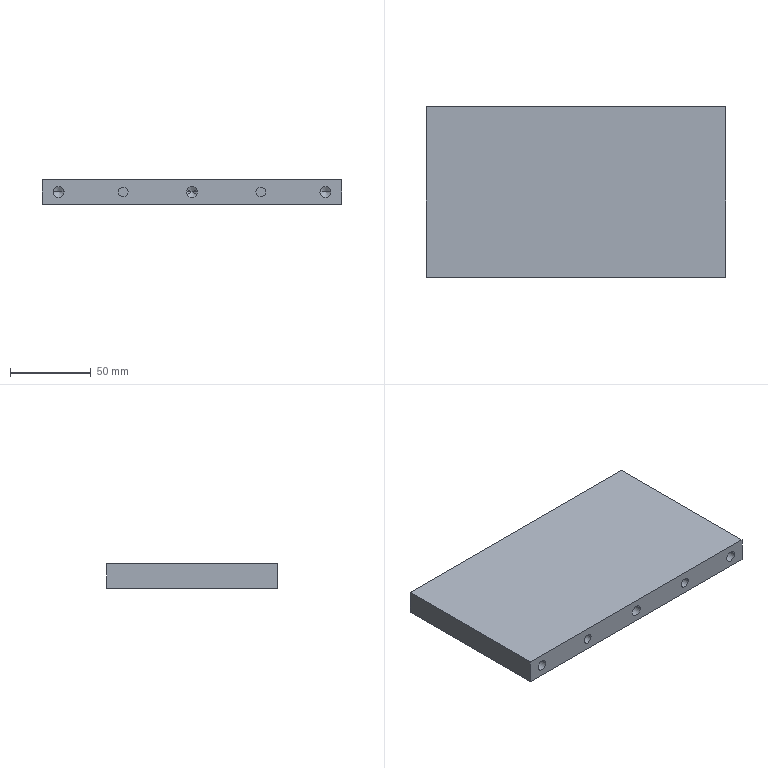Component | SolidWorks | FlipMechanismB-10-1 | 1 solid | 42 faces | box 185 x 105.4 x 15 mm | volume 286584 mm3 | cylinder 20 | cone 12 | plane 10 | commonest cylinder face diameters 6.8 x12 6 x8
STEP:
#1=CARTESIAN_POINT('',(-2.677,-1.323,1.555));
#2=VERTEX_POINT('',#1);
#3=CARTESIAN_POINT('',(-2.441,-1.323,1.555));
#4=VERTEX_POINT('',#3);
#5=CARTESIAN_POINT('',(-2.559,-1.323,1.555));
#6=DIRECTION('',(-0.,-1.,0.));
#7=DIRECTION('',(1.,0.,0.));
#8=AXIS2_PLACEMENT_3D('',#5,#6,#7);
#9=CIRCLE('',#8,0.1181);
#10=EDGE_CURVE('',#2,#4,#9,.T.);
#11=ORIENTED_EDGE('',*,*,#10,.F.);
#12=CARTESIAN_POINT('',(-2.677,-1.559,1.555));
#13=VERTEX_POINT('',#12);
#14=CARTESIAN_POINT('',(-2.677,-1.323,1.555));
#15=DIRECTION('',(-0.,-1.,0.));
#16=VECTOR('',#15,39.37);
#17=LINE('',#14,#16);
#18=EDGE_CURVE('',#2,#13,#17,.T.);
#19=ORIENTED_EDGE('',*,*,#18,.T.);
#20=CARTESIAN_POINT('',(-2.441,-1.559,1.555));
#21=VERTEX_POINT('',#20);
#22=CARTESIAN_POINT('',(-2.559,-1.559,1.555));
#23=DIRECTION('',(-0.,-1.,0.));
#24=DIRECTION('',(1.,0.,0.));
#25=AXIS2_PLACEMENT_3D('',#22,#23,#24);
#26=CIRCLE('',#25,0.1181);
#27=EDGE_CURVE('',#13,#21,#26,.T.);
#28=ORIENTED_EDGE('',*,*,#27,.T.);
#29=CARTESIAN_POINT('',(-2.441,-1.323,1.555));
#30=DIRECTION('',(-0.,-1.,0.));
#31=VECTOR('',#30,39.37);
#32=LINE('',#29,#31);
#33=EDGE_CURVE('',#4,#21,#32,.T.);
#34=ORIENTED_EDGE('',*,*,#33,.F.);
#35=EDGE_LOOP('',(#11,#19,#28,#34));
#36=FACE_OUTER_BOUND('',#35,.T.);
#37=CARTESIAN_POINT('',(-2.559,-1.323,1.555));
#38=DIRECTION('',(-0.,-1.,0.));
#39=DIRECTION('',(1.,0.,0.));
#40=AXIS2_PLACEMENT_3D('',#37,#38,#39);
#41=CYLINDRICAL_SURFACE('',#40,0.1181);
#42=ADVANCED_FACE('',(#36),#41,.F.);
#43=CARTESIAN_POINT('',(0.6693,-1.323,1.555));
#44=VERTEX_POINT('',#43);
#45=CARTESIAN_POINT('',(0.9055,-1.323,1.555));
#46=VERTEX_POINT('',#45);
#47=CARTESIAN_POINT('',(0.7874,-1.323,1.555));
#48=DIRECTION('',(-0.,-1.,0.));
#49=DIRECTION('',(1.,0.,0.));
#50=AXIS2_PLACEMENT_3D('',#47,#48,#49);
#51=CIRCLE('',#50,0.1181);
#52=EDGE_CURVE('',#44,#46,#51,.T.);
#53=ORIENTED_EDGE('',*,*,#52,.F.);
#54=CARTESIAN_POINT('',(0.6693,-1.559,1.555));
#55=VERTEX_POINT('',#54);
#56=CARTESIAN_POINT('',(0.6693,-1.323,1.555));
#57=DIRECTION('',(-0.,-1.,0.));
#58=VECTOR('',#57,39.37);
#59=LINE('',#56,#58);
#60=EDGE_CURVE('',#44,#55,#59,.T.);
#61=ORIENTED_EDGE('',*,*,#60,.T.);
#62=CARTESIAN_POINT('',(0.9055,-1.559,1.555));
#63=VERTEX_POINT('',#62);
#64=CARTESIAN_POINT('',(0.7874,-1.559,1.555));
#65=DIRECTION('',(-0.,-1.,0.));
#66=DIRECTION('',(1.,0.,0.));
#67=AXIS2_PLACEMENT_3D('',#64,#65,#66);
#68=CIRCLE('',#67,0.1181);
#69=EDGE_CURVE('',#55,#63,#68,.T.);
#70=ORIENTED_EDGE('',*,*,#69,.T.);
#71=CARTESIAN_POINT('',(0.9055,-1.323,1.555));
#72=DIRECTION('',(-0.,-1.,0.));
#73=VECTOR('',#72,39.37);
#74=LINE('',#71,#73);
#75=EDGE_CURVE('',#46,#63,#74,.T.);
#76=ORIENTED_EDGE('',*,*,#75,.F.);
#77=EDGE_LOOP('',(#53,#61,#70,#76));
#78=FACE_OUTER_BOUND('',#77,.T.);
#79=CARTESIAN_POINT('',(0.7874,-1.323,1.555));
#80=DIRECTION('',(-0.,-1.,0.));
#81=DIRECTION('',(1.,0.,0.));
#82=AXIS2_PLACEMENT_3D('',#79,#80,#81);
#83=CYLINDRICAL_SURFACE('',#82,0.1181);
#84=ADVANCED_FACE('',(#78),#83,.F.);
#85=CARTESIAN_POINT('',(2.228,-0.6831,1.555));
#86=VERTEX_POINT('',#85);
#87=CARTESIAN_POINT('',(2.496,-0.6831,1.555));
#88=VERTEX_POINT('',#87);
#89=CARTESIAN_POINT('',(2.362,-0.6831,1.555));
#90=DIRECTION('',(-0.,-1.,0.));
#91=DIRECTION('',(1.,0.,0.));
#92=AXIS2_PLACEMENT_3D('',#89,#90,#91);
#93=CIRCLE('',#92,0.1339);
#94=EDGE_CURVE('',#86,#88,#93,.T.);
#95=ORIENTED_EDGE('',*,*,#94,.F.);
#96=CARTESIAN_POINT('',(2.228,-1.559,1.555));
#97=VERTEX_POINT('',#96);
#98=CARTESIAN_POINT('',(2.228,-1.559,1.555));
#99=DIRECTION('',(-0.,-1.,0.));
#100=VECTOR('',#99,39.37);
#101=LINE('',#98,#100);
#102=EDGE_CURVE('',#86,#97,#101,.T.);
#103=ORIENTED_EDGE('',*,*,#102,.T.);
#104=CARTESIAN_POINT('',(2.496,-1.559,1.555));
#105=VERTEX_POINT('',#104);
#106=CARTESIAN_POINT('',(2.362,-1.559,1.555));
#107=DIRECTION('',(-0.,-1.,0.));
#108=DIRECTION('',(1.,0.,0.));
#109=AXIS2_PLACEMENT_3D('',#106,#107,#108);
#110=CIRCLE('',#109,0.1339);
#111=EDGE_CURVE('',#97,#105,#110,.T.);
#112=ORIENTED_EDGE('',*,*,#111,.T.);
#113=CARTESIAN_POINT('',(2.496,-1.559,1.555));
#114=DIRECTION('',(-0.,-1.,0.));
#115=VECTOR('',#114,39.37);
#116=LINE('',#113,#115);
#117=EDGE_CURVE('',#88,#105,#116,.T.);
#118=ORIENTED_EDGE('',*,*,#117,.F.);
#119=EDGE_LOOP('',(#95,#103,#112,#118));
#120=FACE_OUTER_BOUND('',#119,.T.);
#121=CARTESIAN_POINT('',(2.362,-1.559,1.555));
#122=DIRECTION('',(-0.,-1.,0.));
#123=DIRECTION('',(1.,0.,0.));
#124=AXIS2_PLACEMENT_3D('',#121,#122,#123);
#125=CYLINDRICAL_SURFACE('',#124,0.1339);
#126=ADVANCED_FACE('',(#120),#125,.F.);
#127=CARTESIAN_POINT('',(2.362,-0.6026,1.555));
#128=VERTEX_POINT('',#127);
#129=CARTESIAN_POINT('',(2.496,-0.6831,1.555));
#130=DIRECTION('',(0.8572,-0.515,0.));
#131=VECTOR('',#130,39.37);
#132=LINE('',#129,#131);
#133=EDGE_CURVE('',#128,#88,#132,.T.);
#134=ORIENTED_EDGE('',*,*,#133,.F.);
#135=CARTESIAN_POINT('',(2.228,-0.6831,1.555));
#136=DIRECTION('',(-0.8572,-0.515,0.));
#137=VECTOR('',#136,39.37);
#138=LINE('',#135,#137);
#139=EDGE_CURVE('',#128,#86,#138,.T.);
#140=ORIENTED_EDGE('',*,*,#139,.T.);
#141=ORIENTED_EDGE('',*,*,#94,.T.);
#142=EDGE_LOOP('',(#134,#140,#141));
#143=FACE_OUTER_BOUND('',#142,.T.);
#144=CARTESIAN_POINT('',(2.362,-0.6831,1.555));
#145=DIRECTION('',(-0.,-1.,0.));
#146=DIRECTION('',(1.,0.,0.));
#147=AXIS2_PLACEMENT_3D('',#144,#145,#146);
#148=CONICAL_SURFACE('',#147,0.1339,1.03);
#149=ADVANCED_FACE('',(#143),#148,.F.);
#150=CARTESIAN_POINT('',(-1.02,-0.6831,1.555));
#151=VERTEX_POINT('',#150);
#152=CARTESIAN_POINT('',(-0.752,-0.6831,1.555));
#153=VERTEX_POINT('',#152);
#154=CARTESIAN_POINT('',(-0.8858,-0.6831,1.555));
#155=DIRECTION('',(-0.,-1.,0.));
#156=DIRECTION('',(1.,0.,0.));
#157=AXIS2_PLACEMENT_3D('',#154,#155,#156);
#158=CIRCLE('',#157,0.1339);
#159=EDGE_CURVE('',#151,#153,#158,.T.);
#160=ORIENTED_EDGE('',*,*,#159,.F.);
#161=CARTESIAN_POINT('',(-1.02,-1.559,1.555));
#162=VERTEX_POINT('',#161);
#163=CARTESIAN_POINT('',(-1.02,-1.559,1.555));
#164=DIRECTION('',(-0.,-1.,0.));
#165=VECTOR('',#164,39.37);
#166=LINE('',#163,#165);
#167=EDGE_CURVE('',#151,#162,#166,.T.);
#168=ORIENTED_EDGE('',*,*,#167,.T.);
#169=CARTESIAN_POINT('',(-0.752,-1.559,1.555));
#170=VERTEX_POINT('',#169);
#171=CARTESIAN_POINT('',(-0.8858,-1.559,1.555));
#172=DIRECTION('',(-0.,-1.,0.));
#173=DIRECTION('',(1.,0.,0.));
#174=AXIS2_PLACEMENT_3D('',#171,#172,#173);
#175=CIRCLE('',#174,0.1339);
#176=EDGE_CURVE('',#162,#170,#175,.T.);
#177=ORIENTED_EDGE('',*,*,#176,.T.);
#178=CARTESIAN_POINT('',(-0.752,-1.559,1.555));
#179=DIRECTION('',(-0.,-1.,0.));
#180=VECTOR('',#179,39.37);
#181=LINE('',#178,#180);
#182=EDGE_CURVE('',#153,#170,#181,.T.);
#183=ORIENTED_EDGE('',*,*,#182,.F.);
#184=EDGE_LOOP('',(#160,#168,#177,#183));
#185=FACE_OUTER_BOUND('',#184,.T.);
#186=CARTESIAN_POINT('',(-0.8858,-1.559,1.555));
#187=DIRECTION('',(-0.,-1.,0.));
#188=DIRECTION('',(1.,0.,0.));
#189=AXIS2_PLACEMENT_3D('',#186,#187,#188);
#190=CYLINDRICAL_SURFACE('',#189,0.1339);
#191=ADVANCED_FACE('',(#185),#190,.F.);
#192=CARTESIAN_POINT('',(-0.8858,-0.6026,1.555));
#193=VERTEX_POINT('',#192);
#194=CARTESIAN_POINT('',(-0.752,-0.6831,1.555));
#195=DIRECTION('',(0.8572,-0.515,0.));
#196=VECTOR('',#195,39.37);
#197=LINE('',#194,#196);
#198=EDGE_CURVE('',#193,#153,#197,.T.);
#199=ORIENTED_EDGE('',*,*,#198,.F.);
#200=CARTESIAN_POINT('',(-1.02,-0.6831,1.555));
#201=DIRECTION('',(-0.8572,-0.515,0.));
#202=VECTOR('',#201,39.37);
#203=LINE('',#200,#202);
#204=EDGE_CURVE('',#193,#151,#203,.T.);
#205=ORIENTED_EDGE('',*,*,#204,.T.);
#206=ORIENTED_EDGE('',*,*,#159,.T.);
#207=EDGE_LOOP('',(#199,#205,#206));
#208=FACE_OUTER_BOUND('',#207,.T.);
#209=CARTESIAN_POINT('',(-0.8858,-0.6831,1.555));
#210=DIRECTION('',(-0.,-1.,0.));
#211=DIRECTION('',(1.,0.,0.));
#212=AXIS2_PLACEMENT_3D('',#209,#210,#211);
#213=CONICAL_SURFACE('',#212,0.1339,1.03);
#214=ADVANCED_FACE('',(#208),#213,.F.);
#215=CARTESIAN_POINT('',(-4.268,-0.6831,1.555));
#216=VERTEX_POINT('',#215);
#217=CARTESIAN_POINT('',(-4.,-0.6831,1.555));
#218=VERTEX_POINT('',#217);
#219=CARTESIAN_POINT('',(-4.134,-0.6831,1.555));
#220=DIRECTION('',(-0.,-1.,0.));
#221=DIRECTION('',(1.,0.,0.));
#222=AXIS2_PLACEMENT_3D('',#219,#220,#221);
#223=CIRCLE('',#222,0.1339);
#224=EDGE_CURVE('',#216,#218,#223,.T.);
#225=ORIENTED_EDGE('',*,*,#224,.F.);
#226=CARTESIAN_POINT('',(-4.268,-1.559,1.555));
#227=VERTEX_POINT('',#226);
#228=CARTESIAN_POINT('',(-4.268,-1.559,1.555));
#229=DIRECTION('',(-0.,-1.,0.));
#230=VECTOR('',#229,39.37);
#231=LINE('',#228,#230);
#232=EDGE_CURVE('',#216,#227,#231,.T.);
#233=ORIENTED_EDGE('',*,*,#232,.T.);
#234=CARTESIAN_POINT('',(-4.,-1.559,1.555));
#235=VERTEX_POINT('',#234);
#236=CARTESIAN_POINT('',(-4.134,-1.559,1.555));
#237=DIRECTION('',(-0.,-1.,0.));
#238=DIRECTION('',(1.,0.,0.));
#239=AXIS2_PLACEMENT_3D('',#236,#237,#238);
#240=CIRCLE('',#239,0.1339);
#241=EDGE_CURVE('',#227,#235,#240,.T.);
#242=ORIENTED_EDGE('',*,*,#241,.T.);
#243=CARTESIAN_POINT('',(-4.,-1.559,1.555));
#244=DIRECTION('',(-0.,-1.,0.));
#245=VECTOR('',#244,39.37);
#246=LINE('',#243,#245);
#247=EDGE_CURVE('',#218,#235,#246,.T.);
#248=ORIENTED_EDGE('',*,*,#247,.F.);
#249=EDGE_LOOP('',(#225,#233,#242,#248));
#250=FACE_OUTER_BOUND('',#249,.T.);
#251=CARTESIAN_POINT('',(-4.134,-1.559,1.555));
#252=DIRECTION('',(-0.,-1.,0.));
#253=DIRECTION('',(1.,0.,0.));
#254=AXIS2_PLACEMENT_3D('',#251,#252,#253);
#255=CYLINDRICAL_SURFACE('',#254,0.1339);
#256=ADVANCED_FACE('',(#250),#255,.F.);
#257=CARTESIAN_POINT('',(-4.134,-0.6026,1.555));
#258=VERTEX_POINT('',#257);
#259=CARTESIAN_POINT('',(-4.,-0.6831,1.555));
#260=DIRECTION('',(0.8572,-0.515,0.));
#261=VECTOR('',#260,39.37);
#262=LINE('',#259,#261);
#263=EDGE_CURVE('',#258,#218,#262,.T.);
#264=ORIENTED_EDGE('',*,*,#263,.F.);
#265=CARTESIAN_POINT('',(-4.268,-0.6831,1.555));
#266=DIRECTION('',(-0.8572,-0.515,0.));
#267=VECTOR('',#266,39.37);
#268=LINE('',#265,#267);
#269=EDGE_CURVE('',#258,#216,#268,.T.);
#270=ORIENTED_EDGE('',*,*,#269,.T.);
#271=ORIENTED_EDGE('',*,*,#224,.T.);
#272=EDGE_LOOP('',(#264,#270,#271));
#273=FACE_OUTER_BOUND('',#272,.T.);
#274=CARTESIAN_POINT('',(-4.134,-0.6831,1.555));
#275=DIRECTION('',(-0.,-1.,0.));
#276=DIRECTION('',(1.,0.,0.));
#277=AXIS2_PLACEMENT_3D('',#274,#275,#276);
#278=CONICAL_SURFACE('',#277,0.1339,1.03);
#279=ADVANCED_FACE('',(#273),#278,.F.);
#280=CARTESIAN_POINT('',(0.9055,2.197,1.555));
#281=VERTEX_POINT('',#280);
#282=CARTESIAN_POINT('',(0.6693,2.197,1.555));
#283=VERTEX_POINT('',#282);
#284=CARTESIAN_POINT('',(0.7874,2.197,1.555));
#285=DIRECTION('',(0.,1.,-0.));
#286=DIRECTION('',(-1.,0.,0.));
#287=AXIS2_PLACEMENT_3D('',#284,#285,#286);
#288=CIRCLE('',#287,0.1181);
#289=EDGE_CURVE('',#281,#283,#288,.T.);
#290=ORIENTED_EDGE('',*,*,#289,.F.);
#291=CARTESIAN_POINT('',(0.9055,2.591,1.555));
#292=VERTEX_POINT('',#291);
#293=CARTESIAN_POINT('',(0.9055,2.197,1.555));
#294=DIRECTION('',(0.,1.,-0.));
#295=VECTOR('',#294,39.37);
#296=LINE('',#293,#295);
#297=EDGE_CURVE('',#281,#292,#296,.T.);
#298=ORIENTED_EDGE('',*,*,#297,.T.);
#299=CARTESIAN_POINT('',(0.6693,2.591,1.555));
#300=VERTEX_POINT('',#299);
#301=CARTESIAN_POINT('',(0.7874,2.591,1.555));
#302=DIRECTION('',(0.,1.,-0.));
#303=DIRECTION('',(-1.,0.,0.));
#304=AXIS2_PLACEMENT_3D('',#301,#302,#303);
#305=CIRCLE('',#304,0.1181);
#306=EDGE_CURVE('',#292,#300,#305,.T.);
#307=ORIENTED_EDGE('',*,*,#306,.T.);
#308=CARTESIAN_POINT('',(0.6693,2.197,1.555));
#309=DIRECTION('',(0.,1.,-0.));
#310=VECTOR('',#309,39.37);
#311=LINE('',#308,#310);
#312=EDGE_CURVE('',#283,#300,#311,.T.);
#313=ORIENTED_EDGE('',*,*,#312,.F.);
#314=EDGE_LOOP('',(#290,#298,#307,#313));
#315=FACE_OUTER_BOUND('',#314,.T.);
#316=CARTESIAN_POINT('',(0.7874,2.197,1.555));
#317=DIRECTION('',(0.,1.,-0.));
#318=DIRECTION('',(-1.,0.,0.));
#319=AXIS2_PLACEMENT_3D('',#316,#317,#318);
#320=CYLINDRICAL_SURFACE('',#319,0.1181);
#321=ADVANCED_FACE('',(#315),#320,.F.);
#322=CARTESIAN_POINT('',(-2.441,2.197,1.555));
#323=VERTEX_POINT('',#322);
#324=CARTESIAN_POINT('',(-2.677,2.197,1.555));
#325=VERTEX_POINT('',#324);
#326=CARTESIAN_POINT('',(-2.559,2.197,1.555));
#327=DIRECTION('',(0.,1.,-0.));
#328=DIRECTION('',(-1.,0.,0.));
#329=AXIS2_PLACEMENT_3D('',#326,#327,#328);
#330=CIRCLE('',#329,0.1181);
#331=EDGE_CURVE('',#323,#325,#330,.T.);
#332=ORIENTED_EDGE('',*,*,#331,.F.);
#333=CARTESIAN_POINT('',(-2.441,2.591,1.555));
#334=VERTEX_POINT('',#333);
#335=CARTESIAN_POINT('',(-2.441,2.197,1.555));
#336=DIRECTION('',(0.,1.,-0.));
#337=VECTOR('',#336,39.37);
#338=LINE('',#335,#337);
#339=EDGE_CURVE('',#323,#334,#338,.T.);
#340=ORIENTED_EDGE('',*,*,#339,.T.);
#341=CARTESIAN_POINT('',(-2.677,2.591,1.555));
#342=VERTEX_POINT('',#341);
#343=CARTESIAN_POINT('',(-2.559,2.591,1.555));
#344=DIRECTION('',(0.,1.,-0.));
#345=DIRECTION('',(-1.,0.,0.));
#346=AXIS2_PLACEMENT_3D('',#343,#344,#345);
#347=CIRCLE('',#346,0.1181);
#348=EDGE_CURVE('',#334,#342,#347,.T.);
#349=ORIENTED_EDGE('',*,*,#348,.T.);
#350=CARTESIAN_POINT('',(-2.677,2.197,1.555));
#351=DIRECTION('',(0.,1.,-0.));
#352=VECTOR('',#351,39.37);
#353=LINE('',#350,#352);
#354=EDGE_CURVE('',#325,#342,#353,.T.);
#355=ORIENTED_EDGE('',*,*,#354,.F.);
#356=EDGE_LOOP('',(#332,#340,#349,#355));
#357=FACE_OUTER_BOUND('',#356,.T.);
#358=CARTESIAN_POINT('',(-2.559,2.197,1.555));
#359=DIRECTION('',(0.,1.,-0.));
#360=DIRECTION('',(-1.,0.,0.));
#361=AXIS2_PLACEMENT_3D('',#358,#359,#360);
#362=CYLINDRICAL_SURFACE('',#361,0.1181);
#363=ADVANCED_FACE('',(#357),#362,.F.);
#364=CARTESIAN_POINT('',(-4.,1.715,1.555));
#365=VERTEX_POINT('',#364);
#366=CARTESIAN_POINT('',(-4.268,1.715,1.555));
#367=VERTEX_POINT('',#366);
#368=CARTESIAN_POINT('',(-4.134,1.715,1.555));
#369=DIRECTION('',(0.,1.,-0.));
#370=DIRECTION('',(-1.,0.,0.));
#371=AXIS2_PLACEMENT_3D('',#368,#369,#370);
#372=CIRCLE('',#371,0.1339);
#373=EDGE_CURVE('',#365,#367,#372,.T.);
#374=ORIENTED_EDGE('',*,*,#373,.F.);
#375=CARTESIAN_POINT('',(-4.,2.591,1.555));
#376=VERTEX_POINT('',#375);
#377=CARTESIAN_POINT('',(-4.,2.591,1.555));
#378=DIRECTION('',(0.,1.,-0.));
#379=VECTOR('',#378,39.37);
#380=LINE('',#377,#379);
#381=EDGE_CURVE('',#365,#376,#380,.T.);
#382=ORIENTED_EDGE('',*,*,#381,.T.);
#383=CARTESIAN_POINT('',(-4.268,2.591,1.555));
#384=VERTEX_POINT('',#383);
#385=CARTESIAN_POINT('',(-4.134,2.591,1.555));
#386=DIRECTION('',(0.,1.,-0.));
#387=DIRECTION('',(-1.,0.,0.));
#388=AXIS2_PLACEMENT_3D('',#385,#386,#387);
#389=CIRCLE('',#388,0.1339);
#390=EDGE_CURVE('',#376,#384,#389,.T.);
#391=ORIENTED_EDGE('',*,*,#390,.T.);
#392=CARTESIAN_POINT('',(-4.268,2.591,1.555));
#393=DIRECTION('',(0.,1.,-0.));
#394=VECTOR('',#393,39.37);
#395=LINE('',#392,#394);
#396=EDGE_CURVE('',#367,#384,#395,.T.);
#397=ORIENTED_EDGE('',*,*,#396,.F.);
#398=EDGE_LOOP('',(#374,#382,#391,#397));
#399=FACE_OUTER_BOUND('',#398,.T.);
#400=CARTESIAN_POINT('',(-4.134,2.591,1.555));
#401=DIRECTION('',(0.,1.,-0.));
#402=DIRECTION('',(-1.,0.,0.));
#403=AXIS2_PLACEMENT_3D('',#400,#401,#402);
#404=CYLINDRICAL_SURFACE('',#403,0.1339);
#405=ADVANCED_FACE('',(#399),#404,.F.);
#406=CARTESIAN_POINT('',(-4.134,1.634,1.555));
#407=VERTEX_POINT('',#406);
#408=CARTESIAN_POINT('',(-4.268,1.715,1.555));
#409=DIRECTION('',(-0.8572,0.515,-0.));
#410=VECTOR('',#409,39.37);
#411=LINE('',#408,#410);
#412=EDGE_CURVE('',#407,#367,#411,.T.);
#413=ORIENTED_EDGE('',*,*,#412,.F.);
#414=CARTESIAN_POINT('',(-4.,1.715,1.555));
#415=DIRECTION('',(0.8572,0.515,0.));
#416=VECTOR('',#415,39.37);
#417=LINE('',#414,#416);
#418=EDGE_CURVE('',#407,#365,#417,.T.);
#419=ORIENTED_EDGE('',*,*,#418,.T.);
#420=ORIENTED_EDGE('',*,*,#373,.T.);
#421=EDGE_LOOP('',(#413,#419,#420));
#422=FACE_OUTER_BOUND('',#421,.T.);
#423=CARTESIAN_POINT('',(-4.134,1.715,1.555));
#424=DIRECTION('',(0.,1.,-0.));
#425=DIRECTION('',(-1.,0.,0.));
#426=AXIS2_PLACEMENT_3D('',#423,#424,#425);
#427=CONICAL_SURFACE('',#426,0.1339,1.03);
#428=ADVANCED_FACE('',(#422),#427,.F.);
#429=CARTESIAN_POINT('',(-0.752,1.715,1.555));
#430=VERTEX_POINT('',#429);
#431=CARTESIAN_POINT('',(-1.02,1.715,1.555));
#432=VERTEX_POINT('',#431);
#433=CARTESIAN_POINT('',(-0.8858,1.715,1.555));
#434=DIRECTION('',(0.,1.,-0.));
#435=DIRECTION('',(-1.,0.,0.));
#436=AXIS2_PLACEMENT_3D('',#433,#434,#435);
#437=CIRCLE('',#436,0.1339);
#438=EDGE_CURVE('',#430,#432,#437,.T.);
#439=ORIENTED_EDGE('',*,*,#438,.F.);
#440=CARTESIAN_POINT('',(-0.752,2.591,1.555));
#441=VERTEX_POINT('',#440);
#442=CARTESIAN_POINT('',(-0.752,2.591,1.555));
#443=DIRECTION('',(0.,1.,-0.));
#444=VECTOR('',#443,39.37);
#445=LINE('',#442,#444);
#446=EDGE_CURVE('',#430,#441,#445,.T.);
#447=ORIENTED_EDGE('',*,*,#446,.T.);
#448=CARTESIAN_POINT('',(-1.02,2.591,1.555));
#449=VERTEX_POINT('',#448);
#450=CARTESIAN_POINT('',(-0.8858,2.591,1.555));
#451=DIRECTION('',(0.,1.,-0.));
#452=DIRECTION('',(-1.,0.,0.));
#453=AXIS2_PLACEMENT_3D('',#450,#451,#452);
#454=CIRCLE('',#453,0.1339);
#455=EDGE_CURVE('',#441,#449,#454,.T.);
#456=ORIENTED_EDGE('',*,*,#455,.T.);
#457=CARTESIAN_POINT('',(-1.02,2.591,1.555));
#458=DIRECTION('',(0.,1.,-0.));
#459=VECTOR('',#458,39.37);
#460=LINE('',#457,#459);
#461=EDGE_CURVE('',#432,#449,#460,.T.);
#462=ORIENTED_EDGE('',*,*,#461,.F.);
#463=EDGE_LOOP('',(#439,#447,#456,#462));
#464=FACE_OUTER_BOUND('',#463,.T.);
#465=CARTESIAN_POINT('',(-0.8858,2.591,1.555));
#466=DIRECTION('',(0.,1.,-0.));
#467=DIRECTION('',(-1.,0.,0.));
#468=AXIS2_PLACEMENT_3D('',#465,#466,#467);
#469=CYLINDRICAL_SURFACE('',#468,0.1339);
#470=ADVANCED_FACE('',(#464),#469,.F.);
#471=CARTESIAN_POINT('',(-0.8858,1.634,1.555));
#472=VERTEX_POINT('',#471);
#473=CARTESIAN_POINT('',(-1.02,1.715,1.555));
#474=DIRECTION('',(-0.8572,0.515,-0.));
#475=VECTOR('',#474,39.37);
#476=LINE('',#473,#475);
#477=EDGE_CURVE('',#472,#432,#476,.T.);
#478=ORIENTED_EDGE('',*,*,#477,.F.);
#479=CARTESIAN_POINT('',(-0.752,1.715,1.555));
#480=DIRECTION('',(0.8572,0.515,0.));
#481=VECTOR('',#480,39.37);
#482=LINE('',#479,#481);
#483=EDGE_CURVE('',#472,#430,#482,.T.);
#484=ORIENTED_EDGE('',*,*,#483,.T.);
#485=ORIENTED_EDGE('',*,*,#438,.T.);
#486=EDGE_LOOP('',(#478,#484,#485));
#487=FACE_OUTER_BOUND('',#486,.T.);
#488=CARTESIAN_POINT('',(-0.8858,1.715,1.555));
#489=DIRECTION('',(0.,1.,-0.));
#490=DIRECTION('',(-1.,0.,0.));
#491=AXIS2_PLACEMENT_3D('',#488,#489,#490);
#492=CONICAL_SURFACE('',#491,0.1339,1.03);
#493=ADVANCED_FACE('',(#487),#492,.F.);
#494=CARTESIAN_POINT('',(2.496,1.715,1.555));
#495=VERTEX_POINT('',#494);
#496=CARTESIAN_POINT('',(2.228,1.715,1.555));
#497=VERTEX_POINT('',#496);
#498=CARTESIAN_POINT('',(2.362,1.715,1.555));
#499=DIRECTION('',(0.,1.,-0.));
#500=DIRECTION('',(-1.,0.,0.));
#501=AXIS2_PLACEMENT_3D('',#498,#499,#500);
#502=CIRCLE('',#501,0.1339);
#503=EDGE_CURVE('',#495,#497,#502,.T.);
#504=ORIENTED_EDGE('',*,*,#503,.F.);
#505=CARTESIAN_POINT('',(2.496,2.591,1.555));
#506=VERTEX_POINT('',#505);
#507=CARTESIAN_POINT('',(2.496,2.591,1.555));
#508=DIRECTION('',(0.,1.,-0.));
#509=VECTOR('',#508,39.37);
#510=LINE('',#507,#509);
#511=EDGE_CURVE('',#495,#506,#510,.T.);
#512=ORIENTED_EDGE('',*,*,#511,.T.);
#513=CARTESIAN_POINT('',(2.228,2.591,1.555));
#514=VERTEX_POINT('',#513);
#515=CARTESIAN_POINT('',(2.362,2.591,1.555));
#516=DIRECTION('',(0.,1.,-0.));
#517=DIRECTION('',(-1.,0.,0.));
#518=AXIS2_PLACEMENT_3D('',#515,#516,#517);
#519=CIRCLE('',#518,0.1339);
#520=EDGE_CURVE('',#506,#514,#519,.T.);
#521=ORIENTED_EDGE('',*,*,#520,.T.);
#522=CARTESIAN_POINT('',(2.228,2.591,1.555));
#523=DIRECTION('',(0.,1.,-0.));
#524=VECTOR('',#523,39.37);
#525=LINE('',#522,#524);
#526=EDGE_CURVE('',#497,#514,#525,.T.);
#527=ORIENTED_EDGE('',*,*,#526,.F.);
#528=EDGE_LOOP('',(#504,#512,#521,#527));
#529=FACE_OUTER_BOUND('',#528,.T.);
#530=CARTESIAN_POINT('',(2.362,2.591,1.555));
#531=DIRECTION('',(0.,1.,-0.));
#532=DIRECTION('',(-1.,0.,0.));
#533=AXIS2_PLACEMENT_3D('',#530,#531,#532);
#534=CYLINDRICAL_SURFACE('',#533,0.1339);
#535=ADVANCED_FACE('',(#529),#534,.F.);
#536=CARTESIAN_POINT('',(2.362,1.634,1.555));
#537=VERTEX_POINT('',#536);
#538=CARTESIAN_POINT('',(2.228,1.715,1.555));
#539=DIRECTION('',(-0.8572,0.515,-0.));
#540=VECTOR('',#539,39.37);
#541=LINE('',#538,#540);
#542=EDGE_CURVE('',#537,#497,#541,.T.);
#543=ORIENTED_EDGE('',*,*,#542,.F.);
#544=CARTESIAN_POINT('',(2.496,1.715,1.555));
#545=DIRECTION('',(0.8572,0.515,0.));
#546=VECTOR('',#545,39.37);
#547=LINE('',#544,#546);
#548=EDGE_CURVE('',#537,#495,#547,.T.);
#549=ORIENTED_EDGE('',*,*,#548,.T.);
#550=ORIENTED_EDGE('',*,*,#503,.T.);
#551=EDGE_LOOP('',(#543,#549,#550));
#552=FACE_OUTER_BOUND('',#551,.T.);
#553=CARTESIAN_POINT('',(2.362,1.715,1.555));
#554=DIRECTION('',(0.,1.,-0.));
#555=DIRECTION('',(-1.,0.,0.));
#556=AXIS2_PLACEMENT_3D('',#553,#554,#555);
#557=CONICAL_SURFACE('',#556,0.1339,1.03);
#558=ADVANCED_FACE('',(#552),#557,.F.);
#559=CARTESIAN_POINT('',(2.756,-1.559,1.26));
#560=VERTEX_POINT('',#559);
#561=CARTESIAN_POINT('',(2.756,2.591,1.26));
#562=VERTEX_POINT('',#561);
#563=CARTESIAN_POINT('',(2.756,-1.559,1.26));
#564=DIRECTION('',(0.,1.,-0.));
#565=VECTOR('',#564,39.37);
#566=LINE('',#563,#565);
#567=EDGE_CURVE('',#560,#562,#566,.T.);
#568=ORIENTED_EDGE('',*,*,#567,.T.);
#569=CARTESIAN_POINT('',(2.756,2.591,1.85));
#570=VERTEX_POINT('',#569);
#571=CARTESIAN_POINT('',(2.756,2.591,1.85));
#572=DIRECTION('',(-0.,-0.,-1.));
#573=VECTOR('',#572,39.37);
#574=LINE('',#571,#573);
#575=EDGE_CURVE('',#570,#562,#574,.T.);
#576=ORIENTED_EDGE('',*,*,#575,.F.);
#577=CARTESIAN_POINT('',(2.756,-1.559,1.85));
#578=VERTEX_POINT('',#577);
#579=CARTESIAN_POINT('',(2.756,-1.559,1.85));
#580=DIRECTION('',(0.,1.,-0.));
#581=VECTOR('',#580,39.37);
#582=LINE('',#579,#581);
#583=EDGE_CURVE('',#578,#570,#582,.T.);
#584=ORIENTED_EDGE('',*,*,#583,.F.);
#585=CARTESIAN_POINT('',(2.756,-1.559,1.85));
#586=DIRECTION('',(-0.,-0.,-1.));
#587=VECTOR('',#586,39.37);
#588=LINE('',#585,#587);
#589=EDGE_CURVE('',#578,#560,#588,.T.);
#590=ORIENTED_EDGE('',*,*,#589,.T.);
#591=EDGE_LOOP('',(#568,#576,#584,#590));
#592=FACE_OUTER_BOUND('',#591,.T.);
#593=CARTESIAN_POINT('',(2.756,-1.559,1.85));
#594=DIRECTION('',(-1.,0.,0.));
#595=DIRECTION('',(-0.,-1.,0.));
#596=AXIS2_PLACEMENT_3D('',#593,#594,#595);
#597=PLANE('',#596);
#598=ADVANCED_FACE('',(#592),#597,.F.);
#599=CARTESIAN_POINT('',(0.7874,2.591,1.555));
#600=DIRECTION('',(0.,1.,-0.));
#601=DIRECTION('',(-1.,0.,0.));
#602=AXIS2_PLACEMENT_3D('',#599,#600,#601);
#603=CIRCLE('',#602,0.1181);
#604=EDGE_CURVE('',#300,#292,#603,.T.);
#605=ORIENTED_EDGE('',*,*,#604,.F.);
#606=ORIENTED_EDGE('',*,*,#306,.F.);
#607=EDGE_LOOP('',(#605,#606));
#608=FACE_BOUND('',#607,.T.);
#609=CARTESIAN_POINT('',(-2.559,2.591,1.555));
#610=DIRECTION('',(0.,1.,-0.));
#611=DIRECTION('',(-1.,0.,0.));
#612=AXIS2_PLACEMENT_3D('',#609,#610,#611);
#613=CIRCLE('',#612,0.1181);
#614=EDGE_CURVE('',#342,#334,#613,.T.);
#615=ORIENTED_EDGE('',*,*,#614,.F.);
#616=ORIENTED_EDGE('',*,*,#348,.F.);
#617=EDGE_LOOP('',(#615,#616));
#618=FACE_BOUND('',#617,.T.);
#619=CARTESIAN_POINT('',(-4.134,2.591,1.555));
#620=DIRECTION('',(0.,1.,-0.));
#621=DIRECTION('',(-1.,0.,0.));
#622=AXIS2_PLACEMENT_3D('',#619,#620,#621);
#623=CIRCLE('',#622,0.1339);
#624=EDGE_CURVE('',#384,#376,#623,.T.);
#625=ORIENTED_EDGE('',*,*,#624,.F.);
#626=ORIENTED_EDGE('',*,*,#390,.F.);
#627=EDGE_LOOP('',(#625,#626));
#628=FACE_BOUND('',#627,.T.);
#629=CARTESIAN_POINT('',(-0.8858,2.591,1.555));
#630=DIRECTION('',(0.,1.,-0.));
#631=DIRECTION('',(-1.,0.,0.));
#632=AXIS2_PLACEMENT_3D('',#629,#630,#631);
#633=CIRCLE('',#632,0.1339);
#634=EDGE_CURVE('',#449,#441,#633,.T.);
#635=ORIENTED_EDGE('',*,*,#634,.F.);
#636=ORIENTED_EDGE('',*,*,#455,.F.);
#637=EDGE_LOOP('',(#635,#636));
#638=FACE_BOUND('',#637,.T.);
#639=CARTESIAN_POINT('',(2.362,2.591,1.555));
#640=DIRECTION('',(0.,1.,-0.));
#641=DIRECTION('',(-1.,0.,0.));
#642=AXIS2_PLACEMENT_3D('',#639,#640,#641);
#643=CIRCLE('',#642,0.1339);
#644=EDGE_CURVE('',#514,#506,#643,.T.);
#645=ORIENTED_EDGE('',*,*,#644,.F.);
#646=ORIENTED_EDGE('',*,*,#520,.F.);
#647=EDGE_LOOP('',(#645,#646));
#648=FACE_BOUND('',#647,.T.);
#649=CARTESIAN_POINT('',(-4.528,2.591,1.26));
#650=VERTEX_POINT('',#649);
#651=CARTESIAN_POINT('',(2.756,2.591,1.26));
#652=DIRECTION('',(-1.,0.,0.));
#653=VECTOR('',#652,39.37);
#654=LINE('',#651,#653);
#655=EDGE_CURVE('',#562,#650,#654,.T.);
#656=ORIENTED_EDGE('',*,*,#655,.T.);
#657=CARTESIAN_POINT('',(-4.528,2.591,1.85));
#658=VERTEX_POINT('',#657);
#659=CARTESIAN_POINT('',(-4.528,2.591,1.85));
#660=DIRECTION('',(-0.,-0.,-1.));
#661=VECTOR('',#660,39.37);
#662=LINE('',#659,#661);
#663=EDGE_CURVE('',#658,#650,#662,.T.);
#664=ORIENTED_EDGE('',*,*,#663,.F.);
#665=CARTESIAN_POINT('',(2.756,2.591,1.85));
#666=DIRECTION('',(-1.,0.,0.));
#667=VECTOR('',#666,39.37);
#668=LINE('',#665,#667);
#669=EDGE_CURVE('',#570,#658,#668,.T.);
#670=ORIENTED_EDGE('',*,*,#669,.F.);
#671=ORIENTED_EDGE('',*,*,#575,.T.);
#672=EDGE_LOOP('',(#656,#664,#670,#671));
#673=FACE_OUTER_BOUND('',#672,.T.);
#674=CARTESIAN_POINT('',(2.756,2.591,1.85));
#675=DIRECTION('',(-0.,-1.,0.));
#676=DIRECTION('',(1.,-0.,0.));
#677=AXIS2_PLACEMENT_3D('',#674,#675,#676);
#678=PLANE('',#677);
#679=ADVANCED_FACE('',(#608,#618,#628,#638,#648,#673),#678,.F.);
#680=CARTESIAN_POINT('',(-4.528,-1.559,1.26));
#681=VERTEX_POINT('',#680);
#682=CARTESIAN_POINT('',(-4.528,-1.559,1.26));
#683=DIRECTION('',(-0.,-1.,0.));
#684=VECTOR('',#683,39.37);
#685=LINE('',#682,#684);
#686=EDGE_CURVE('',#650,#681,#685,.T.);
#687=ORIENTED_EDGE('',*,*,#686,.T.);
#688=CARTESIAN_POINT('',(-4.528,-1.559,1.85));
#689=VERTEX_POINT('',#688);
#690=CARTESIAN_POINT('',(-4.528,-1.559,1.85));
#691=DIRECTION('',(-0.,-0.,-1.));
#692=VECTOR('',#691,39.37);
#693=LINE('',#690,#692);
#694=EDGE_CURVE('',#689,#681,#693,.T.);
#695=ORIENTED_EDGE('',*,*,#694,.F.);
#696=CARTESIAN_POINT('',(-4.528,-1.559,1.85));
#697=DIRECTION('',(-0.,-1.,0.));
#698=VECTOR('',#697,39.37);
#699=LINE('',#696,#698);
#700=EDGE_CURVE('',#658,#689,#699,.T.);
#701=ORIENTED_EDGE('',*,*,#700,.F.);
#702=ORIENTED_EDGE('',*,*,#663,.T.);
#703=EDGE_LOOP('',(#687,#695,#701,#702));
#704=FACE_OUTER_BOUND('',#703,.T.);
#705=CARTESIAN_POINT('',(-4.528,-1.559,1.85));
#706=DIRECTION('',(1.,-0.,0.));
#707=DIRECTION('',(0.,1.,-0.));
#708=AXIS2_PLACEMENT_3D('',#705,#706,#707);
#709=PLANE('',#708);
#710=ADVANCED_FACE('',(#704),#709,.F.);
#711=CARTESIAN_POINT('',(-2.559,-1.559,1.555));
#712=DIRECTION('',(-0.,-1.,0.));
#713=DIRECTION('',(1.,0.,0.));
#714=AXIS2_PLACEMENT_3D('',#711,#712,#713);
#715=CIRCLE('',#714,0.1181);
#716=EDGE_CURVE('',#21,#13,#715,.T.);
#717=ORIENTED_EDGE('',*,*,#716,.F.);
#718=ORIENTED_EDGE('',*,*,#27,.F.);
#719=EDGE_LOOP('',(#717,#718));
#720=FACE_BOUND('',#719,.T.);
#721=CARTESIAN_POINT('',(0.7874,-1.559,1.555));
#722=DIRECTION('',(-0.,-1.,0.));
#723=DIRECTION('',(1.,0.,0.));
#724=AXIS2_PLACEMENT_3D('',#721,#722,#723);
#725=CIRCLE('',#724,0.1181);
#726=EDGE_CURVE('',#63,#55,#725,.T.);
#727=ORIENTED_EDGE('',*,*,#726,.F.);
#728=ORIENTED_EDGE('',*,*,#69,.F.);
#729=EDGE_LOOP('',(#727,#728));
#730=FACE_BOUND('',#729,.T.);
#731=CARTESIAN_POINT('',(2.362,-1.559,1.555));
#732=DIRECTION('',(-0.,-1.,0.));
#733=DIRECTION('',(1.,0.,0.));
#734=AXIS2_PLACEMENT_3D('',#731,#732,#733);
#735=CIRCLE('',#734,0.1339);
#736=EDGE_CURVE('',#105,#97,#735,.T.);
#737=ORIENTED_EDGE('',*,*,#736,.F.);
#738=ORIENTED_EDGE('',*,*,#111,.F.);
#739=EDGE_LOOP('',(#737,#738));
#740=FACE_BOUND('',#739,.T.);
#741=CARTESIAN_POINT('',(-0.8858,-1.559,1.555));
#742=DIRECTION('',(-0.,-1.,0.));
#743=DIRECTION('',(1.,0.,0.));
#744=AXIS2_PLACEMENT_3D('',#741,#742,#743);
#745=CIRCLE('',#744,0.1339);
#746=EDGE_CURVE('',#170,#162,#745,.T.);
#747=ORIENTED_EDGE('',*,*,#746,.F.);
#748=ORIENTED_EDGE('',*,*,#176,.F.);
#749=EDGE_LOOP('',(#747,#748));
#750=FACE_BOUND('',#749,.T.);
#751=CARTESIAN_POINT('',(-4.134,-1.559,1.555));
#752=DIRECTION('',(-0.,-1.,0.));
#753=DIRECTION('',(1.,0.,0.));
#754=AXIS2_PLACEMENT_3D('',#751,#752,#753);
#755=CIRCLE('',#754,0.1339);
#756=EDGE_CURVE('',#235,#227,#755,.T.);
#757=ORIENTED_EDGE('',*,*,#756,.F.);
#758=ORIENTED_EDGE('',*,*,#241,.F.);
#759=EDGE_LOOP('',(#757,#758));
#760=FACE_BOUND('',#759,.T.);
#761=CARTESIAN_POINT('',(2.756,-1.559,1.26));
#762=DIRECTION('',(1.,-0.,0.));
#763=VECTOR('',#762,39.37);
#764=LINE('',#761,#763);
#765=EDGE_CURVE('',#681,#560,#764,.T.);
#766=ORIENTED_EDGE('',*,*,#765,.T.);
#767=ORIENTED_EDGE('',*,*,#589,.F.);
#768=CARTESIAN_POINT('',(2.756,-1.559,1.85));
#769=DIRECTION('',(1.,-0.,0.));
#770=VECTOR('',#769,39.37);
#771=LINE('',#768,#770);
#772=EDGE_CURVE('',#689,#578,#771,.T.);
#773=ORIENTED_EDGE('',*,*,#772,.F.);
#774=ORIENTED_EDGE('',*,*,#694,.T.);
#775=EDGE_LOOP('',(#766,#767,#773,#774));
#776=FACE_OUTER_BOUND('',#775,.T.);
#777=CARTESIAN_POINT('',(2.756,-1.559,1.85));
#778=DIRECTION('',(0.,1.,-0.));
#779=DIRECTION('',(-1.,0.,0.));
#780=AXIS2_PLACEMENT_3D('',#777,#778,#779);
#781=PLANE('',#780);
#782=ADVANCED_FACE('',(#720,#730,#740,#750,#760,#776),#781,.F.);
#783=ORIENTED_EDGE('',*,*,#583,.T.);
#784=ORIENTED_EDGE('',*,*,#669,.T.);
#785=ORIENTED_EDGE('',*,*,#700,.T.);
#786=ORIENTED_EDGE('',*,*,#772,.T.);
#787=EDGE_LOOP('',(#783,#784,#785,#786));
#788=FACE_OUTER_BOUND('',#787,.T.);
#789=CARTESIAN_POINT('',(-0.8858,0.5157,1.85));
#790=DIRECTION('',(0.,0.,1.));
#791=DIRECTION('',(0.,1.,-0.));
#792=AXIS2_PLACEMENT_3D('',#789,#790,#791);
#793=PLANE('',#792);
#794=ADVANCED_FACE('',(#788),#793,.T.);
#795=ORIENTED_EDGE('',*,*,#567,.F.);
#796=ORIENTED_EDGE('',*,*,#765,.F.);
#797=ORIENTED_EDGE('',*,*,#686,.F.);
#798=ORIENTED_EDGE('',*,*,#655,.F.);
#799=EDGE_LOOP('',(#795,#796,#797,#798));
#800=FACE_OUTER_BOUND('',#799,.T.);
#801=CARTESIAN_POINT('',(-0.8858,0.5157,1.26));
#802=DIRECTION('',(0.,0.,1.));
#803=DIRECTION('',(0.,1.,-0.));
#804=AXIS2_PLACEMENT_3D('',#801,#802,#803);
#805=PLANE('',#804);
#806=ADVANCED_FACE('',(#800),#805,.F.);
#807=ORIENTED_EDGE('',*,*,#548,.F.);
#808=ORIENTED_EDGE('',*,*,#542,.T.);
#809=CARTESIAN_POINT('',(2.362,1.715,1.555));
#810=DIRECTION('',(0.,1.,-0.));
#811=DIRECTION('',(-1.,0.,0.));
#812=AXIS2_PLACEMENT_3D('',#809,#810,#811);
#813=CIRCLE('',#812,0.1339);
#814=EDGE_CURVE('',#497,#495,#813,.T.);
#815=ORIENTED_EDGE('',*,*,#814,.T.);
#816=EDGE_LOOP('',(#807,#808,#815));
#817=FACE_OUTER_BOUND('',#816,.T.);
#818=CARTESIAN_POINT('',(2.362,1.715,1.555));
#819=DIRECTION('',(0.,1.,-0.));
#820=DIRECTION('',(-1.,0.,0.));
#821=AXIS2_PLACEMENT_3D('',#818,#819,#820);
#822=CONICAL_SURFACE('',#821,0.1339,1.03);
#823=ADVANCED_FACE('',(#817),#822,.F.);
#824=ORIENTED_EDGE('',*,*,#511,.F.);
#825=ORIENTED_EDGE('',*,*,#814,.F.);
#826=ORIENTED_EDGE('',*,*,#526,.T.);
#827=ORIENTED_EDGE('',*,*,#644,.T.);
#828=EDGE_LOOP('',(#824,#825,#826,#827));
#829=FACE_OUTER_BOUND('',#828,.T.);
#830=CARTESIAN_POINT('',(2.362,2.591,1.555));
#831=DIRECTION('',(0.,1.,-0.));
#832=DIRECTION('',(-1.,0.,0.));
#833=AXIS2_PLACEMENT_3D('',#830,#831,#832);
#834=CYLINDRICAL_SURFACE('',#833,0.1339);
#835=ADVANCED_FACE('',(#829),#834,.F.);
#836=ORIENTED_EDGE('',*,*,#483,.F.);
#837=ORIENTED_EDGE('',*,*,#477,.T.);
#838=CARTESIAN_POINT('',(-0.8858,1.715,1.555));
#839=DIRECTION('',(0.,1.,-0.));
#840=DIRECTION('',(-1.,0.,0.));
#841=AXIS2_PLACEMENT_3D('',#838,#839,#840);
#842=CIRCLE('',#841,0.1339);
#843=EDGE_CURVE('',#432,#430,#842,.T.);
#844=ORIENTED_EDGE('',*,*,#843,.T.);
#845=EDGE_LOOP('',(#836,#837,#844));
#846=FACE_OUTER_BOUND('',#845,.T.);
#847=CARTESIAN_POINT('',(-0.8858,1.715,1.555));
#848=DIRECTION('',(0.,1.,-0.));
#849=DIRECTION('',(-1.,0.,0.));
#850=AXIS2_PLACEMENT_3D('',#847,#848,#849);
#851=CONICAL_SURFACE('',#850,0.1339,1.03);
#852=ADVANCED_FACE('',(#846),#851,.F.);
#853=ORIENTED_EDGE('',*,*,#446,.F.);
#854=ORIENTED_EDGE('',*,*,#843,.F.);
#855=ORIENTED_EDGE('',*,*,#461,.T.);
#856=ORIENTED_EDGE('',*,*,#634,.T.);
#857=EDGE_LOOP('',(#853,#854,#855,#856));
#858=FACE_OUTER_BOUND('',#857,.T.);
#859=CARTESIAN_POINT('',(-0.8858,2.591,1.555));
#860=DIRECTION('',(0.,1.,-0.));
#861=DIRECTION('',(-1.,0.,0.));
#862=AXIS2_PLACEMENT_3D('',#859,#860,#861);
#863=CYLINDRICAL_SURFACE('',#862,0.1339);
#864=ADVANCED_FACE('',(#858),#863,.F.);
#865=ORIENTED_EDGE('',*,*,#418,.F.);
#866=ORIENTED_EDGE('',*,*,#412,.T.);
#867=CARTESIAN_POINT('',(-4.134,1.715,1.555));
#868=DIRECTION('',(0.,1.,-0.));
#869=DIRECTION('',(-1.,0.,0.));
#870=AXIS2_PLACEMENT_3D('',#867,#868,#869);
#871=CIRCLE('',#870,0.1339);
#872=EDGE_CURVE('',#367,#365,#871,.T.);
#873=ORIENTED_EDGE('',*,*,#872,.T.);
#874=EDGE_LOOP('',(#865,#866,#873));
#875=FACE_OUTER_BOUND('',#874,.T.);
#876=CARTESIAN_POINT('',(-4.134,1.715,1.555));
#877=DIRECTION('',(0.,1.,-0.));
#878=DIRECTION('',(-1.,0.,0.));
#879=AXIS2_PLACEMENT_3D('',#876,#877,#878);
#880=CONICAL_SURFACE('',#879,0.1339,1.03);
#881=ADVANCED_FACE('',(#875),#880,.F.);
#882=ORIENTED_EDGE('',*,*,#381,.F.);
#883=ORIENTED_EDGE('',*,*,#872,.F.);
#884=ORIENTED_EDGE('',*,*,#396,.T.);
#885=ORIENTED_EDGE('',*,*,#624,.T.);
#886=EDGE_LOOP('',(#882,#883,#884,#885));
#887=FACE_OUTER_BOUND('',#886,.T.);
#888=CARTESIAN_POINT('',(-4.134,2.591,1.555));
#889=DIRECTION('',(0.,1.,-0.));
#890=DIRECTION('',(-1.,0.,0.));
#891=AXIS2_PLACEMENT_3D('',#888,#889,#890);
#892=CYLINDRICAL_SURFACE('',#891,0.1339);
#893=ADVANCED_FACE('',(#887),#892,.F.);
#894=ORIENTED_EDGE('',*,*,#339,.F.);
#895=CARTESIAN_POINT('',(-2.559,2.197,1.555));
#896=DIRECTION('',(0.,1.,-0.));
#897=DIRECTION('',(-1.,0.,0.));
#898=AXIS2_PLACEMENT_3D('',#895,#896,#897);
#899=CIRCLE('',#898,0.1181);
#900=EDGE_CURVE('',#325,#323,#899,.T.);
#901=ORIENTED_EDGE('',*,*,#900,.F.);
#902=ORIENTED_EDGE('',*,*,#354,.T.);
#903=ORIENTED_EDGE('',*,*,#614,.T.);
#904=EDGE_LOOP('',(#894,#901,#902,#903));
#905=FACE_OUTER_BOUND('',#904,.T.);
#906=CARTESIAN_POINT('',(-2.559,2.197,1.555));
#907=DIRECTION('',(0.,1.,-0.));
#908=DIRECTION('',(-1.,0.,0.));
#909=AXIS2_PLACEMENT_3D('',#906,#907,#908);
#910=CYLINDRICAL_SURFACE('',#909,0.1181);
#911=ADVANCED_FACE('',(#905),#910,.F.);
#912=ORIENTED_EDGE('',*,*,#900,.T.);
#913=ORIENTED_EDGE('',*,*,#331,.T.);
#914=EDGE_LOOP('',(#912,#913));
#915=FACE_OUTER_BOUND('',#914,.T.);
#916=CARTESIAN_POINT('',(-2.559,2.197,1.555));
#917=DIRECTION('',(0.,1.,-0.));
#918=DIRECTION('',(-1.,0.,0.));
#919=AXIS2_PLACEMENT_3D('',#916,#917,#918);
#920=PLANE('',#919);
#921=ADVANCED_FACE('',(#915),#920,.T.);
#922=ORIENTED_EDGE('',*,*,#297,.F.);
#923=CARTESIAN_POINT('',(0.7874,2.197,1.555));
#924=DIRECTION('',(0.,1.,-0.));
#925=DIRECTION('',(-1.,0.,0.));
#926=AXIS2_PLACEMENT_3D('',#923,#924,#925);
#927=CIRCLE('',#926,0.1181);
#928=EDGE_CURVE('',#283,#281,#927,.T.);
#929=ORIENTED_EDGE('',*,*,#928,.F.);
#930=ORIENTED_EDGE('',*,*,#312,.T.);
#931=ORIENTED_EDGE('',*,*,#604,.T.);
#932=EDGE_LOOP('',(#922,#929,#930,#931));
#933=FACE_OUTER_BOUND('',#932,.T.);
#934=CARTESIAN_POINT('',(0.7874,2.197,1.555));
#935=DIRECTION('',(0.,1.,-0.));
#936=DIRECTION('',(-1.,0.,0.));
#937=AXIS2_PLACEMENT_3D('',#934,#935,#936);
#938=CYLINDRICAL_SURFACE('',#937,0.1181);
#939=ADVANCED_FACE('',(#933),#938,.F.);
#940=ORIENTED_EDGE('',*,*,#928,.T.);
#941=ORIENTED_EDGE('',*,*,#289,.T.);
#942=EDGE_LOOP('',(#940,#941));
#943=FACE_OUTER_BOUND('',#942,.T.);
#944=CARTESIAN_POINT('',(0.7874,2.197,1.555));
#945=DIRECTION('',(0.,1.,-0.));
#946=DIRECTION('',(-1.,0.,0.));
#947=AXIS2_PLACEMENT_3D('',#944,#945,#946);
#948=PLANE('',#947);
#949=ADVANCED_FACE('',(#943),#948,.T.);
#950=ORIENTED_EDGE('',*,*,#269,.F.);
#951=ORIENTED_EDGE('',*,*,#263,.T.);
#952=CARTESIAN_POINT('',(-4.134,-0.6831,1.555));
#953=DIRECTION('',(-0.,-1.,0.));
#954=DIRECTION('',(1.,0.,0.));
#955=AXIS2_PLACEMENT_3D('',#952,#953,#954);
#956=CIRCLE('',#955,0.1339);
#957=EDGE_CURVE('',#218,#216,#956,.T.);
#958=ORIENTED_EDGE('',*,*,#957,.T.);
#959=EDGE_LOOP('',(#950,#951,#958));
#960=FACE_OUTER_BOUND('',#959,.T.);
#961=CARTESIAN_POINT('',(-4.134,-0.6831,1.555));
#962=DIRECTION('',(-0.,-1.,0.));
#963=DIRECTION('',(1.,0.,0.));
#964=AXIS2_PLACEMENT_3D('',#961,#962,#963);
#965=CONICAL_SURFACE('',#964,0.1339,1.03);
#966=ADVANCED_FACE('',(#960),#965,.F.);
#967=ORIENTED_EDGE('',*,*,#232,.F.);
#968=ORIENTED_EDGE('',*,*,#957,.F.);
#969=ORIENTED_EDGE('',*,*,#247,.T.);
#970=ORIENTED_EDGE('',*,*,#756,.T.);
#971=EDGE_LOOP('',(#967,#968,#969,#970));
#972=FACE_OUTER_BOUND('',#971,.T.);
#973=CARTESIAN_POINT('',(-4.134,-1.559,1.555));
#974=DIRECTION('',(-0.,-1.,0.));
#975=DIRECTION('',(1.,0.,0.));
#976=AXIS2_PLACEMENT_3D('',#973,#974,#975);
#977=CYLINDRICAL_SURFACE('',#976,0.1339);
#978=ADVANCED_FACE('',(#972),#977,.F.);
#979=ORIENTED_EDGE('',*,*,#204,.F.);
#980=ORIENTED_EDGE('',*,*,#198,.T.);
#981=CARTESIAN_POINT('',(-0.8858,-0.6831,1.555));
#982=DIRECTION('',(-0.,-1.,0.));
#983=DIRECTION('',(1.,0.,0.));
#984=AXIS2_PLACEMENT_3D('',#981,#982,#983);
#985=CIRCLE('',#984,0.1339);
#986=EDGE_CURVE('',#153,#151,#985,.T.);
#987=ORIENTED_EDGE('',*,*,#986,.T.);
#988=EDGE_LOOP('',(#979,#980,#987));
#989=FACE_OUTER_BOUND('',#988,.T.);
#990=CARTESIAN_POINT('',(-0.8858,-0.6831,1.555));
#991=DIRECTION('',(-0.,-1.,0.));
#992=DIRECTION('',(1.,0.,0.));
#993=AXIS2_PLACEMENT_3D('',#990,#991,#992);
#994=CONICAL_SURFACE('',#993,0.1339,1.03);
#995=ADVANCED_FACE('',(#989),#994,.F.);
#996=ORIENTED_EDGE('',*,*,#167,.F.);
#997=ORIENTED_EDGE('',*,*,#986,.F.);
#998=ORIENTED_EDGE('',*,*,#182,.T.);
#999=ORIENTED_EDGE('',*,*,#746,.T.);
#1000=EDGE_LOOP('',(#996,#997,#998,#999));
#1001=FACE_OUTER_BOUND('',#1000,.T.);
#1002=CARTESIAN_POINT('',(-0.8858,-1.559,1.555));
#1003=DIRECTION('',(-0.,-1.,0.));
#1004=DIRECTION('',(1.,0.,0.));
#1005=AXIS2_PLACEMENT_3D('',#1002,#1003,#1004);
#1006=CYLINDRICAL_SURFACE('',#1005,0.1339);
#1007=ADVANCED_FACE('',(#1001),#1006,.F.);
#1008=ORIENTED_EDGE('',*,*,#139,.F.);
#1009=ORIENTED_EDGE('',*,*,#133,.T.);
#1010=CARTESIAN_POINT('',(2.362,-0.6831,1.555));
#1011=DIRECTION('',(-0.,-1.,0.));
#1012=DIRECTION('',(1.,0.,0.));
#1013=AXIS2_PLACEMENT_3D('',#1010,#1011,#1012);
#1014=CIRCLE('',#1013,0.1339);
#1015=EDGE_CURVE('',#88,#86,#1014,.T.);
#1016=ORIENTED_EDGE('',*,*,#1015,.T.);
#1017=EDGE_LOOP('',(#1008,#1009,#1016));
#1018=FACE_OUTER_BOUND('',#1017,.T.);
#1019=CARTESIAN_POINT('',(2.362,-0.6831,1.555));
#1020=DIRECTION('',(-0.,-1.,0.));
#1021=DIRECTION('',(1.,0.,0.));
#1022=AXIS2_PLACEMENT_3D('',#1019,#1020,#1021);
#1023=CONICAL_SURFACE('',#1022,0.1339,1.03);
#1024=ADVANCED_FACE('',(#1018),#1023,.F.);
#1025=ORIENTED_EDGE('',*,*,#102,.F.);
#1026=ORIENTED_EDGE('',*,*,#1015,.F.);
#1027=ORIENTED_EDGE('',*,*,#117,.T.);
#1028=ORIENTED_EDGE('',*,*,#736,.T.);
#1029=EDGE_LOOP('',(#1025,#1026,#1027,#1028));
#1030=FACE_OUTER_BOUND('',#1029,.T.);
#1031=CARTESIAN_POINT('',(2.362,-1.559,1.555));
#1032=DIRECTION('',(-0.,-1.,0.));
#1033=DIRECTION('',(1.,0.,0.));
#1034=AXIS2_PLACEMENT_3D('',#1031,#1032,#1033);
#1035=CYLINDRICAL_SURFACE('',#1034,0.1339);
#1036=ADVANCED_FACE('',(#1030),#1035,.F.);
#1037=ORIENTED_EDGE('',*,*,#60,.F.);
#1038=CARTESIAN_POINT('',(0.7874,-1.323,1.555));
#1039=DIRECTION('',(-0.,-1.,0.));
#1040=DIRECTION('',(1.,0.,0.));
#1041=AXIS2_PLACEMENT_3D('',#1038,#1039,#1040);
#1042=CIRCLE('',#1041,0.1181);
#1043=EDGE_CURVE('',#46,#44,#1042,.T.);
#1044=ORIENTED_EDGE('',*,*,#1043,.F.);
#1045=ORIENTED_EDGE('',*,*,#75,.T.);
#1046=ORIENTED_EDGE('',*,*,#726,.T.);
#1047=EDGE_LOOP('',(#1037,#1044,#1045,#1046));
#1048=FACE_OUTER_BOUND('',#1047,.T.);
#1049=CARTESIAN_POINT('',(0.7874,-1.323,1.555));
#1050=DIRECTION('',(-0.,-1.,0.));
#1051=DIRECTION('',(1.,0.,0.));
#1052=AXIS2_PLACEMENT_3D('',#1049,#1050,#1051);
#1053=CYLINDRICAL_SURFACE('',#1052,0.1181);
#1054=ADVANCED_FACE('',(#1048),#1053,.F.);
#1055=ORIENTED_EDGE('',*,*,#1043,.T.);
#1056=ORIENTED_EDGE('',*,*,#52,.T.);
#1057=EDGE_LOOP('',(#1055,#1056));
#1058=FACE_OUTER_BOUND('',#1057,.T.);
#1059=CARTESIAN_POINT('',(0.7874,-1.323,1.555));
#1060=DIRECTION('',(-0.,-1.,0.));
#1061=DIRECTION('',(1.,-0.,0.));
#1062=AXIS2_PLACEMENT_3D('',#1059,#1060,#1061);
#1063=PLANE('',#1062);
#1064=ADVANCED_FACE('',(#1058),#1063,.T.);
#1065=ORIENTED_EDGE('',*,*,#18,.F.);
#1066=CARTESIAN_POINT('',(-2.559,-1.323,1.555));
#1067=DIRECTION('',(-0.,-1.,0.));
#1068=DIRECTION('',(1.,0.,0.));
#1069=AXIS2_PLACEMENT_3D('',#1066,#1067,#1068);
#1070=CIRCLE('',#1069,0.1181);
#1071=EDGE_CURVE('',#4,#2,#1070,.T.);
#1072=ORIENTED_EDGE('',*,*,#1071,.F.);
#1073=ORIENTED_EDGE('',*,*,#33,.T.);
#1074=ORIENTED_EDGE('',*,*,#716,.T.);
#1075=EDGE_LOOP('',(#1065,#1072,#1073,#1074));
#1076=FACE_OUTER_BOUND('',#1075,.T.);
#1077=CARTESIAN_POINT('',(-2.559,-1.323,1.555));
#1078=DIRECTION('',(-0.,-1.,0.));
#1079=DIRECTION('',(1.,0.,0.));
#1080=AXIS2_PLACEMENT_3D('',#1077,#1078,#1079);
#1081=CYLINDRICAL_SURFACE('',#1080,0.1181);
#1082=ADVANCED_FACE('',(#1076),#1081,.F.);
#1083=ORIENTED_EDGE('',*,*,#1071,.T.);
#1084=ORIENTED_EDGE('',*,*,#10,.T.);
#1085=EDGE_LOOP('',(#1083,#1084));
#1086=FACE_OUTER_BOUND('',#1085,.T.);
#1087=CARTESIAN_POINT('',(-2.559,-1.323,1.555));
#1088=DIRECTION('',(-0.,-1.,0.));
#1089=DIRECTION('',(1.,-0.,0.));
#1090=AXIS2_PLACEMENT_3D('',#1087,#1088,#1089);
#1091=PLANE('',#1090);
#1092=ADVANCED_FACE('',(#1086),#1091,.T.);
#1093=CLOSED_SHELL('',(#42,#84,#126,#149,#191,#214,#256,#279,#321,#363,#405,#428,#470,#493,#535,#558,#598,#679,#710,#782,#794,#806,#823,#835,#852,#864,#881,#893,#911,#921,#939,#949,#966,#978,#995,#1007,#1024,#1036,#1054,#1064,#1082,#1092));
#1094=MANIFOLD_SOLID_BREP('',#1093);
#1095=CARTESIAN_POINT('',(0.,0.,0.));
#1096=DIRECTION('',(0.,0.,1.));
#1097=DIRECTION('',(1.,0.,0.));
#1098=AXIS2_PLACEMENT_3D('',#1095,#1096,#1097);
#1099=(LENGTH_UNIT()NAMED_UNIT(*)SI_UNIT($,.METRE.));
#1100=LENGTH_MEASURE_WITH_UNIT(LENGTH_MEASURE(0.0254),#1099);
#1101=DIMENSIONAL_EXPONENTS(1.,0.,0.,0.,0.,0.,0.);
#1102=(CONVERSION_BASED_UNIT('',#1100)LENGTH_UNIT()NAMED_UNIT(#1101));
#1103=UNCERTAINTY_MEASURE_WITH_UNIT(LENGTH_MEASURE(0.00001),#1102,'','');
#1104=(NAMED_UNIT(*)PLANE_ANGLE_UNIT()SI_UNIT($,.RADIAN.));
#1105=(NAMED_UNIT(*)SI_UNIT($,.STERADIAN.)SOLID_ANGLE_UNIT());
#1106=(GEOMETRIC_REPRESENTATION_CONTEXT(3)GLOBAL_UNCERTAINTY_ASSIGNED_CONTEXT((#1103))GLOBAL_UNIT_ASSIGNED_CONTEXT((#1102,#1104,#1105))REPRESENTATION_CONTEXT('',''));
#1107=ADVANCED_BREP_SHAPE_REPRESENTATION('',(#1094,#1098),#1106);
#1108=COLOUR_RGB('',0.7922,0.8196,0.9333);
#1109=FILL_AREA_STYLE_COLOUR('',#1108);
#1110=FILL_AREA_STYLE('',(#1109));
#1111=SURFACE_STYLE_FILL_AREA(#1110);
#1112=SURFACE_SIDE_STYLE('',(#1111));
#1113=SURFACE_STYLE_USAGE(.BOTH.,#1112);
#1114=PRESENTATION_STYLE_ASSIGNMENT((#1113));
#1115=STYLED_ITEM('',(#1114),#1094);
#1116=PRESENTATION_LAYER_ASSIGNMENT('','',(#1115));
#1117=(LENGTH_UNIT()NAMED_UNIT(*)SI_UNIT($,.METRE.));
#1118=LENGTH_MEASURE_WITH_UNIT(LENGTH_MEASURE(0.0254),#1117);
#1119=DIMENSIONAL_EXPONENTS(1.,0.,0.,0.,0.,0.,0.);
#1120=(CONVERSION_BASED_UNIT('',#1118)LENGTH_UNIT()NAMED_UNIT(#1119));
#1121=UNCERTAINTY_MEASURE_WITH_UNIT(LENGTH_MEASURE(0.00001),#1120,'','');
#1122=(NAMED_UNIT(*)PLANE_ANGLE_UNIT()SI_UNIT($,.RADIAN.));
#1123=(NAMED_UNIT(*)SI_UNIT($,.STERADIAN.)SOLID_ANGLE_UNIT());
#1124=(GEOMETRIC_REPRESENTATION_CONTEXT(3)GLOBAL_UNCERTAINTY_ASSIGNED_CONTEXT((#1121))GLOBAL_UNIT_ASSIGNED_CONTEXT((#1120,#1122,#1123))REPRESENTATION_CONTEXT('',''));
#1125=MECHANICAL_DESIGN_GEOMETRIC_PRESENTATION_REPRESENTATION('',(#1115),#1124);